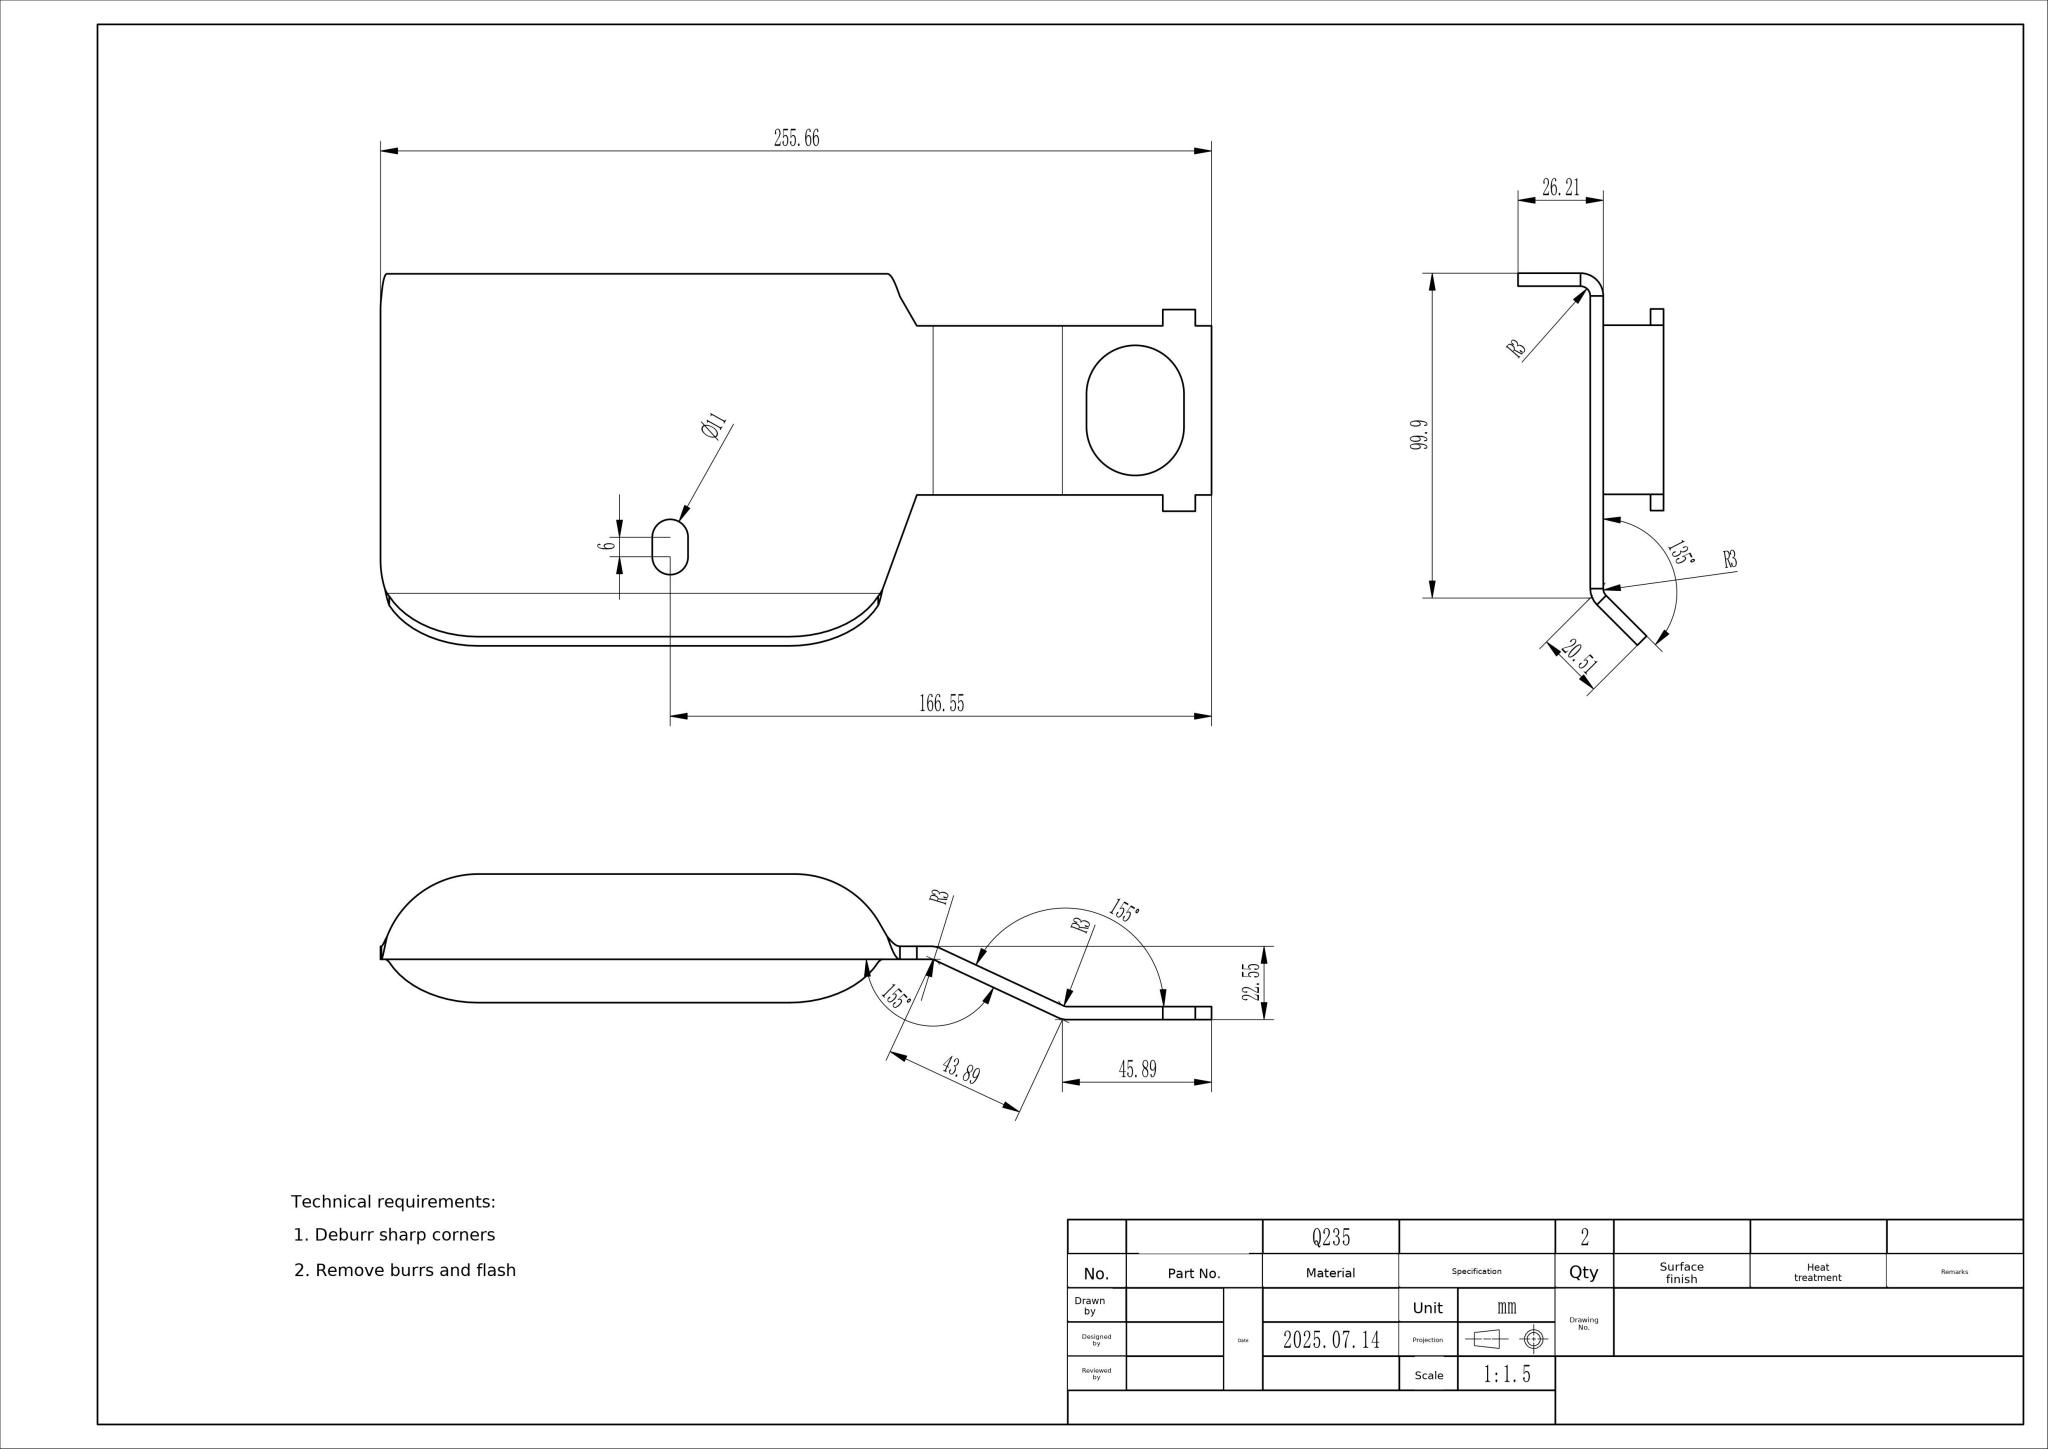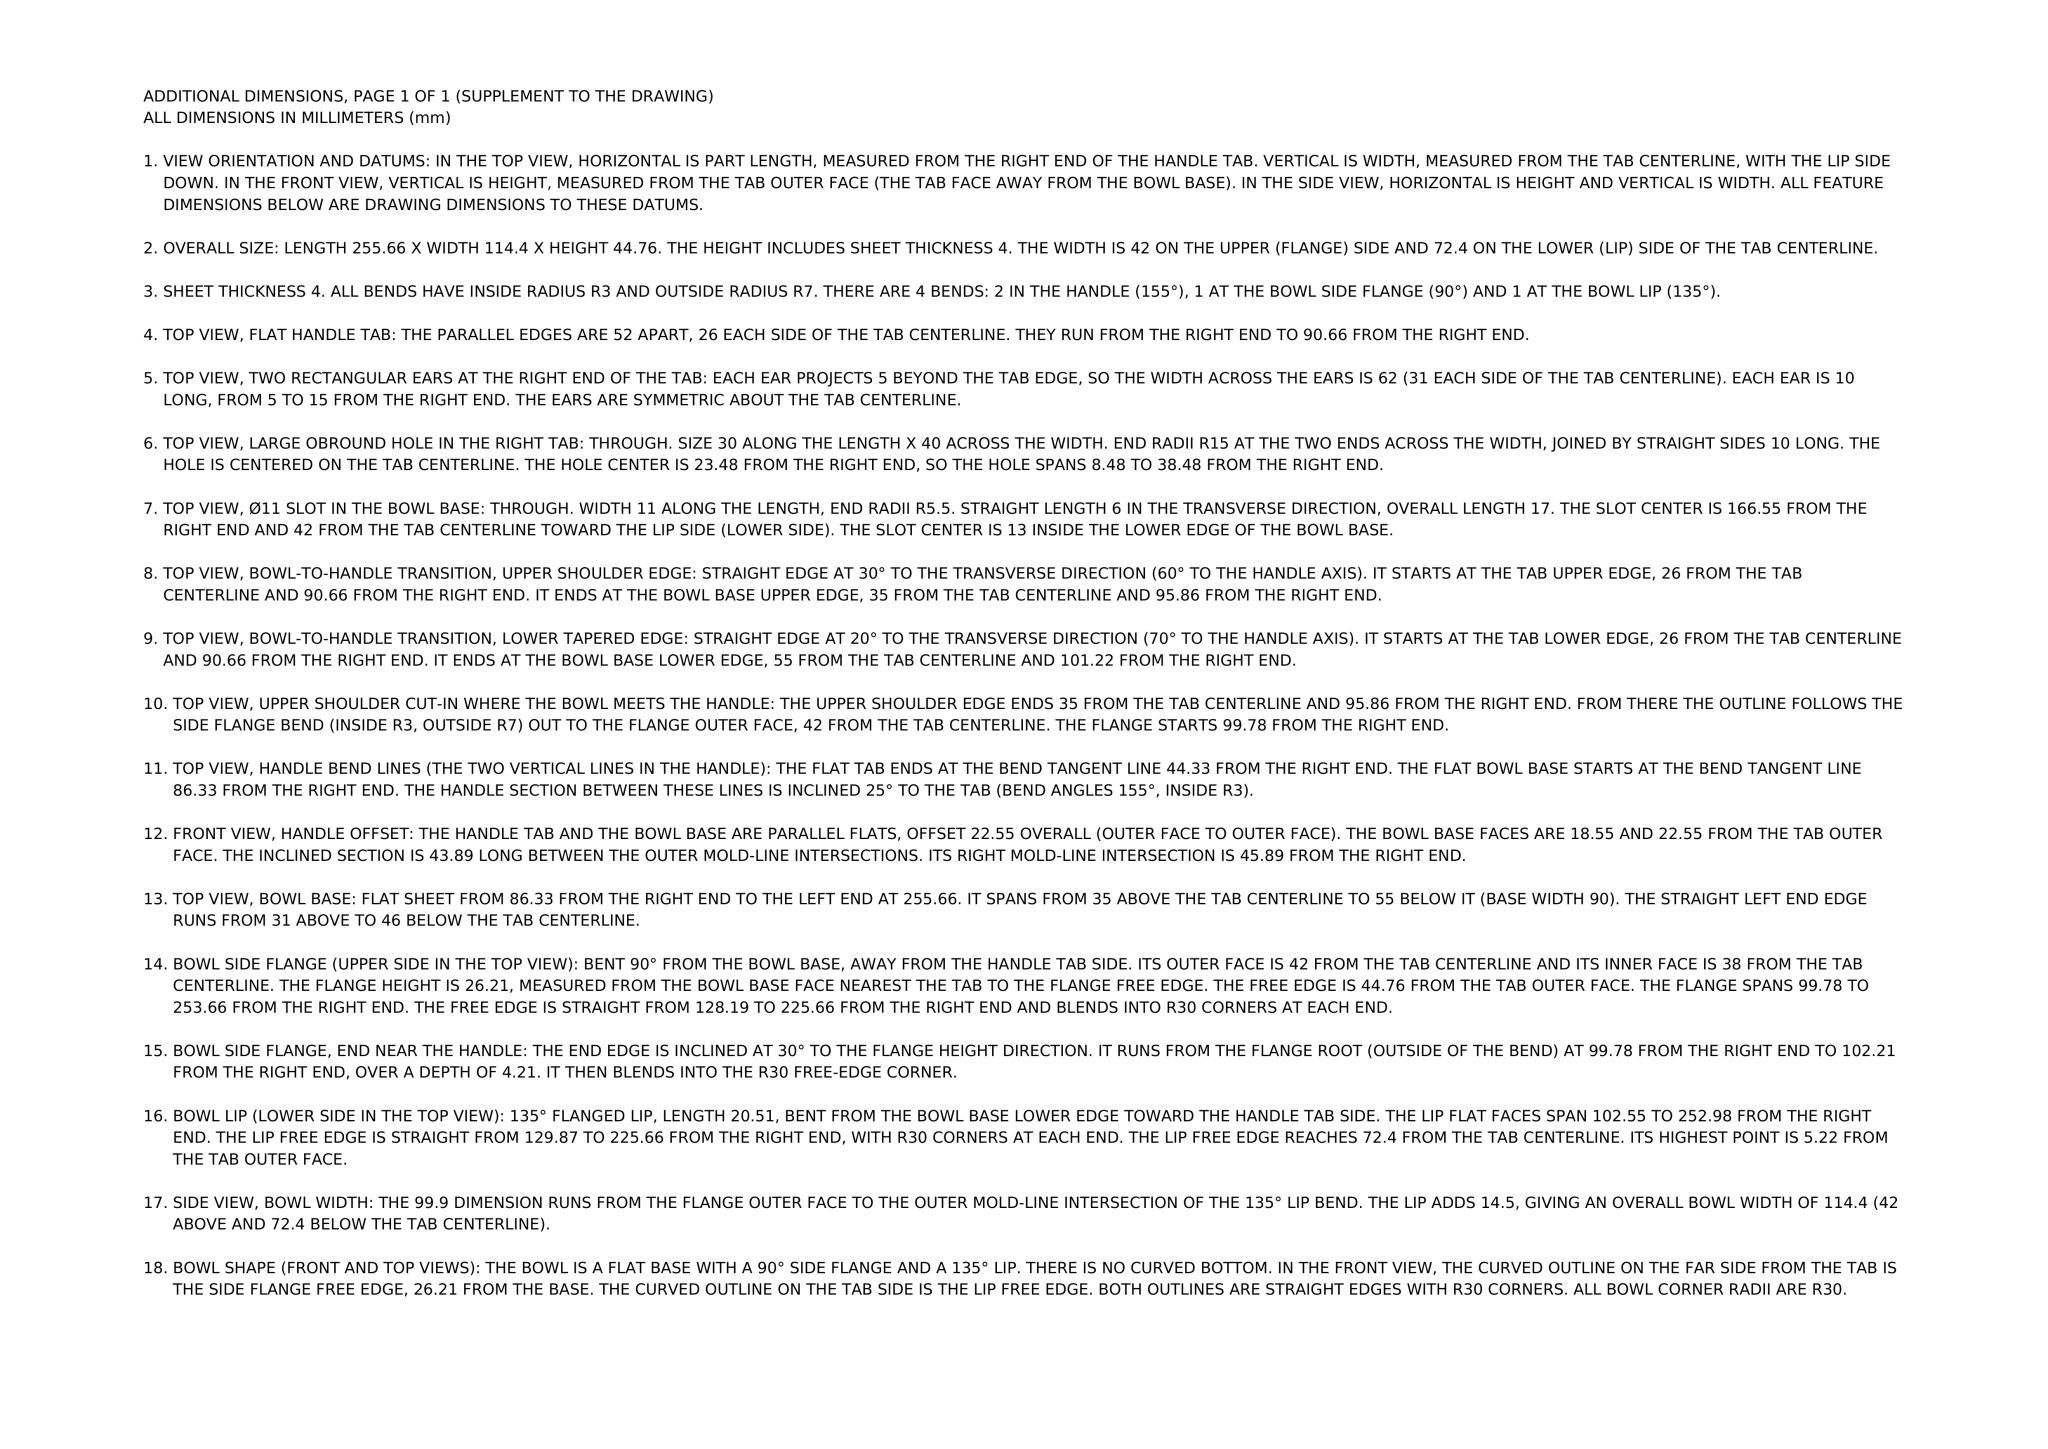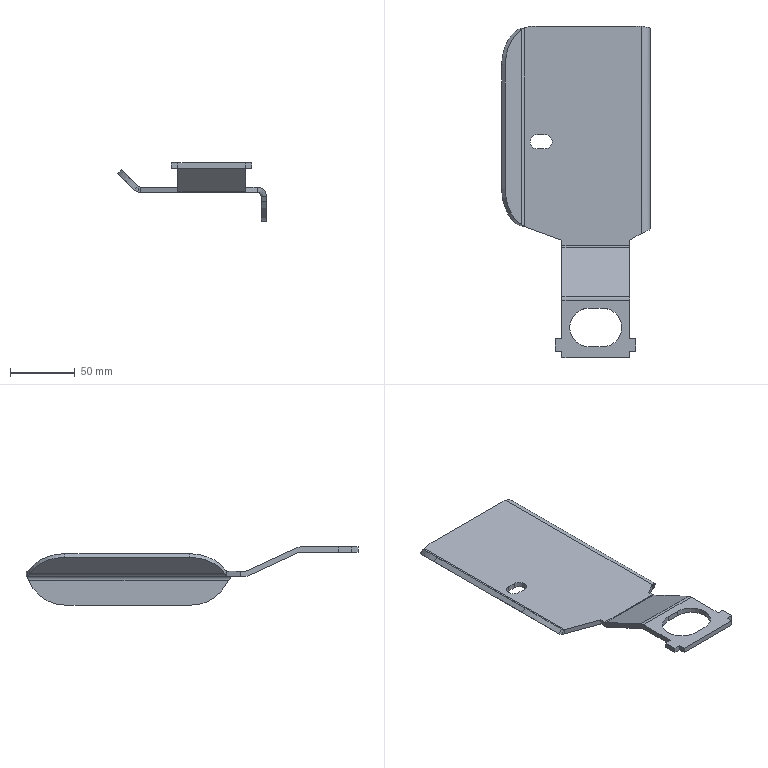Part | NX | mm | 1 solid | 54 faces | box 114.4 x 255.66 x 44.76 mm | volume 101546 mm3 | plane 31 | cylinder 18 | spline 5 | commonest cylinder face diameters 60 x6 14 x4 6 x4 11 x2 30 x2